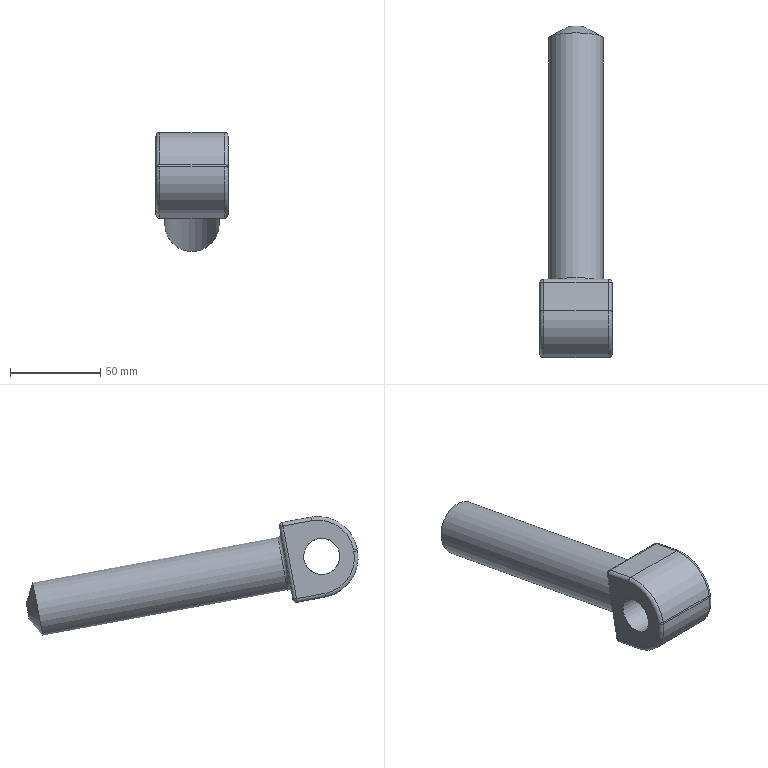Component | NX | CCJ-011 | 1 solid | 34 faces | volume 112874 mm3 | cylinder 16 | plane 8 | torus 5 | sphere 4 | cone 1 | commonest cylinder face diameters 4 x10 20 x2 44 x2 30 x1 10 x1